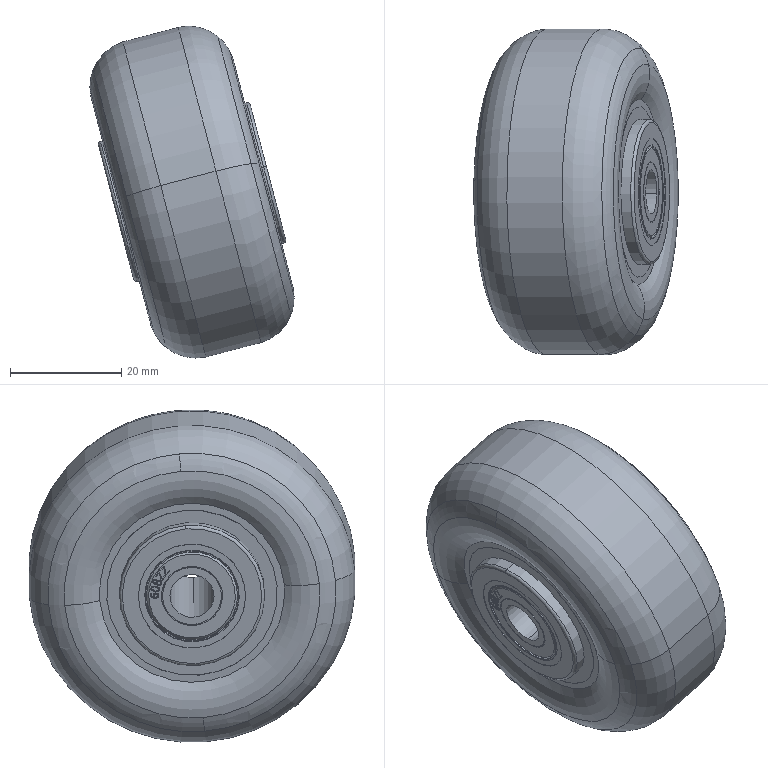Component | SolidWorks | PC-CAJ-P08-1_Rueda 2 in AZUL-1_Pieza1-1 | 1 solid | 155 faces | volume 64306 mm3 | spline 50 | plane 49 | cylinder 28 | torus 16 | cone 12 | commonest cylinder face diameters 11 x4 16.4 x4 10.6 x4 19.3 x4 26.1 x4 30.7 x4 7.92 x2 58.72 x2 | material Plain Carbon Steel